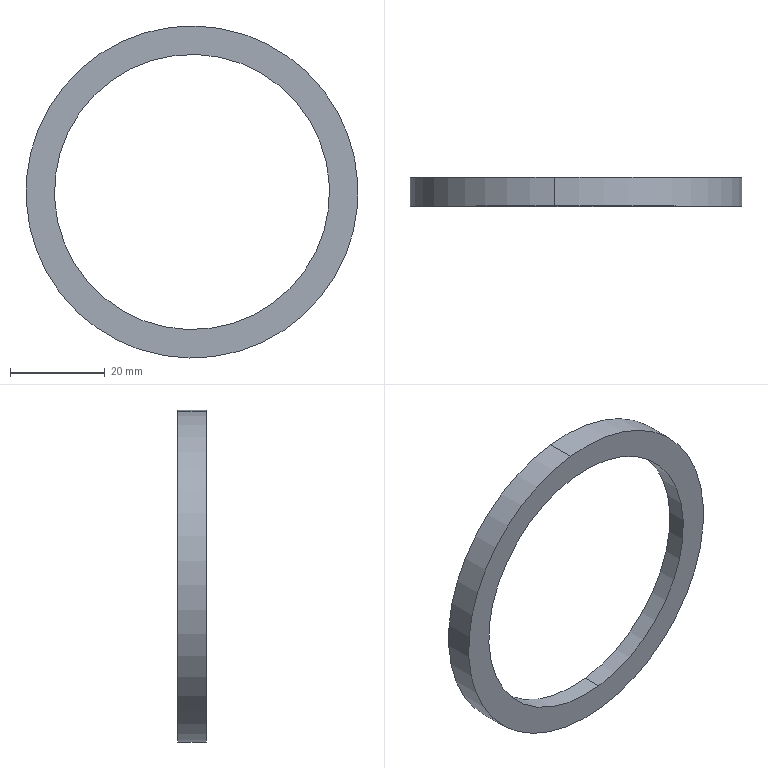Component | SolidWorks | Assembly4.1-1_118.1-1 | 1 solid | 9 faces | box 70 x 6 x 70 mm | volume 6088 mm3 | cylinder 6 | plane 3 | commonest cylinder face diameters 64 x2 70 x2 58 x2
build123d program:
from build123d import *

# Parameters (mm, degrees)
SKETCH1_R           = 35
SKETCH1_R_2         = 29
BOSS_EXTRUDE1_DEPTH = 6
SKETCH2_R           = 32
CUT_EXTRUDE1_DEPTH  = 2


with BuildPart() as part:
    # Sketch1 → Boss-Extrude1 (new body)
    with BuildSketch(Plane.XY):
        Circle(SKETCH1_R)
        Circle(SKETCH1_R_2, mode=Mode.SUBTRACT)
    extrude(amount=BOSS_EXTRUDE1_DEPTH)

    # Sketch2 → Cut-Extrude1 (cut)
    with BuildSketch(Plane.XY.offset(6)):
        Circle(SKETCH2_R)
    extrude(amount=-CUT_EXTRUDE1_DEPTH, mode=Mode.SUBTRACT)


solid = part.part

# Placed as in the assembly
solid = solid.moved(Location((0, -39.5, -0.4), (-90, 0, 0)))
STEP:
#1=COLOUR_RGB('',0.7922,0.8196,0.9333);
#2=FILL_AREA_STYLE_COLOUR('',#1);
#3=FILL_AREA_STYLE('',(#2));
#4=SURFACE_STYLE_FILL_AREA(#3);
#5=SURFACE_SIDE_STYLE('',(#4));
#6=SURFACE_STYLE_USAGE(.BOTH.,#5);
#7=PRESENTATION_STYLE_ASSIGNMENT((#6));
#8=CARTESIAN_POINT('',(-0.1653,-1.398,1.233));
#9=VERTEX_POINT('',#8);
#10=CARTESIAN_POINT('',(0.1653,-1.398,-1.265));
#11=VERTEX_POINT('',#10);
#12=CARTESIAN_POINT('',(-0.,-1.398,-0.01575));
#13=DIRECTION('',(0.,1.,-0.));
#14=DIRECTION('',(0.1312,0.,-0.9914));
#15=AXIS2_PLACEMENT_3D('',#12,#13,#14);
#16=CIRCLE('',#15,1.26);
#17=EDGE_CURVE('',#9,#11,#16,.T.);
#18=ORIENTED_EDGE('',*,*,#17,.F.);
#19=CARTESIAN_POINT('',(-0.1653,-1.319,1.233));
#20=VERTEX_POINT('',#19);
#21=CARTESIAN_POINT('',(-0.1653,-1.398,1.233));
#22=DIRECTION('',(0.,1.,-0.));
#23=VECTOR('',#22,39.37);
#24=LINE('',#21,#23);
#25=EDGE_CURVE('',#9,#20,#24,.T.);
#26=ORIENTED_EDGE('',*,*,#25,.T.);
#27=CARTESIAN_POINT('',(0.1653,-1.319,-1.265));
#28=VERTEX_POINT('',#27);
#29=CARTESIAN_POINT('',(-0.,-1.319,-0.01575));
#30=DIRECTION('',(0.,1.,-0.));
#31=DIRECTION('',(0.1312,0.,-0.9914));
#32=AXIS2_PLACEMENT_3D('',#29,#30,#31);
#33=CIRCLE('',#32,1.26);
#34=EDGE_CURVE('',#20,#28,#33,.T.);
#35=ORIENTED_EDGE('',*,*,#34,.T.);
#36=CARTESIAN_POINT('',(0.1653,-1.398,-1.265));
#37=DIRECTION('',(0.,1.,-0.));
#38=VECTOR('',#37,39.37);
#39=LINE('',#36,#38);
#40=EDGE_CURVE('',#11,#28,#39,.T.);
#41=ORIENTED_EDGE('',*,*,#40,.F.);
#42=EDGE_LOOP('',(#18,#26,#35,#41));
#43=FACE_OUTER_BOUND('',#42,.T.);
#44=CARTESIAN_POINT('',(-0.,-1.398,-0.01575));
#45=DIRECTION('',(0.,1.,-0.));
#46=DIRECTION('',(0.1312,0.,-0.9914));
#47=AXIS2_PLACEMENT_3D('',#44,#45,#46);
#48=CYLINDRICAL_SURFACE('',#47,1.26);
#49=ADVANCED_FACE('',(#43),#48,.F.);
#50=CARTESIAN_POINT('',(0.1808,-1.319,-1.382));
#51=VERTEX_POINT('',#50);
#52=CARTESIAN_POINT('',(-0.1808,-1.319,1.35));
#53=VERTEX_POINT('',#52);
#54=CARTESIAN_POINT('',(-0.,-1.319,-0.01575));
#55=DIRECTION('',(0.,1.,-0.));
#56=DIRECTION('',(0.1312,0.,-0.9914));
#57=AXIS2_PLACEMENT_3D('',#54,#55,#56);
#58=CIRCLE('',#57,1.378);
#59=EDGE_CURVE('',#51,#53,#58,.T.);
#60=ORIENTED_EDGE('',*,*,#59,.F.);
#61=CARTESIAN_POINT('',(0.1808,-1.555,-1.382));
#62=VERTEX_POINT('',#61);
#63=CARTESIAN_POINT('',(0.1808,-1.319,-1.382));
#64=DIRECTION('',(-0.,-1.,0.));
#65=VECTOR('',#64,39.37);
#66=LINE('',#63,#65);
#67=EDGE_CURVE('',#51,#62,#66,.T.);
#68=ORIENTED_EDGE('',*,*,#67,.T.);
#69=CARTESIAN_POINT('',(-0.1808,-1.555,1.35));
#70=VERTEX_POINT('',#69);
#71=CARTESIAN_POINT('',(-0.,-1.555,-0.01575));
#72=DIRECTION('',(0.,1.,-0.));
#73=DIRECTION('',(0.1312,0.,-0.9914));
#74=AXIS2_PLACEMENT_3D('',#71,#72,#73);
#75=CIRCLE('',#74,1.378);
#76=EDGE_CURVE('',#62,#70,#75,.T.);
#77=ORIENTED_EDGE('',*,*,#76,.T.);
#78=CARTESIAN_POINT('',(-0.1808,-1.319,1.35));
#79=DIRECTION('',(-0.,-1.,0.));
#80=VECTOR('',#79,39.37);
#81=LINE('',#78,#80);
#82=EDGE_CURVE('',#53,#70,#81,.T.);
#83=ORIENTED_EDGE('',*,*,#82,.F.);
#84=EDGE_LOOP('',(#60,#68,#77,#83));
#85=FACE_OUTER_BOUND('',#84,.T.);
#86=CARTESIAN_POINT('',(-0.,-1.319,-0.01575));
#87=DIRECTION('',(-0.,-1.,0.));
#88=DIRECTION('',(-0.1312,0.,0.9914));
#89=AXIS2_PLACEMENT_3D('',#86,#87,#88);
#90=CYLINDRICAL_SURFACE('',#89,1.378);
#91=ADVANCED_FACE('',(#85),#90,.T.);
#92=CARTESIAN_POINT('',(-0.1498,-1.398,1.116));
#93=VERTEX_POINT('',#92);
#94=CARTESIAN_POINT('',(0.1498,-1.398,-1.148));
#95=VERTEX_POINT('',#94);
#96=CARTESIAN_POINT('',(-0.,-1.398,-0.01575));
#97=DIRECTION('',(0.,1.,-0.));
#98=DIRECTION('',(0.1312,0.,-0.9914));
#99=AXIS2_PLACEMENT_3D('',#96,#97,#98);
#100=CIRCLE('',#99,1.142);
#101=EDGE_CURVE('',#93,#95,#100,.T.);
#102=ORIENTED_EDGE('',*,*,#101,.T.);
#103=CARTESIAN_POINT('',(0.1498,-1.555,-1.148));
#104=VERTEX_POINT('',#103);
#105=CARTESIAN_POINT('',(0.1498,-1.319,-1.148));
#106=DIRECTION('',(-0.,-1.,0.));
#107=VECTOR('',#106,39.37);
#108=LINE('',#105,#107);
#109=EDGE_CURVE('',#95,#104,#108,.T.);
#110=ORIENTED_EDGE('',*,*,#109,.T.);
#111=CARTESIAN_POINT('',(-0.1498,-1.555,1.116));
#112=VERTEX_POINT('',#111);
#113=CARTESIAN_POINT('',(-0.,-1.555,-0.01575));
#114=DIRECTION('',(0.,1.,-0.));
#115=DIRECTION('',(0.1312,0.,-0.9914));
#116=AXIS2_PLACEMENT_3D('',#113,#114,#115);
#117=CIRCLE('',#116,1.142);
#118=EDGE_CURVE('',#112,#104,#117,.T.);
#119=ORIENTED_EDGE('',*,*,#118,.F.);
#120=CARTESIAN_POINT('',(-0.1498,-1.319,1.116));
#121=DIRECTION('',(-0.,-1.,0.));
#122=VECTOR('',#121,39.37);
#123=LINE('',#120,#122);
#124=EDGE_CURVE('',#93,#112,#123,.T.);
#125=ORIENTED_EDGE('',*,*,#124,.F.);
#126=EDGE_LOOP('',(#102,#110,#119,#125));
#127=FACE_OUTER_BOUND('',#126,.T.);
#128=CARTESIAN_POINT('',(-0.,-1.319,-0.01575));
#129=DIRECTION('',(-0.,-1.,0.));
#130=DIRECTION('',(-0.1312,0.,0.9914));
#131=AXIS2_PLACEMENT_3D('',#128,#129,#130);
#132=CYLINDRICAL_SURFACE('',#131,1.142);
#133=ADVANCED_FACE('',(#127),#132,.F.);
#134=ORIENTED_EDGE('',*,*,#109,.F.);
#135=CARTESIAN_POINT('',(-0.,-1.398,-0.01575));
#136=DIRECTION('',(0.,1.,-0.));
#137=DIRECTION('',(0.1312,0.,-0.9914));
#138=AXIS2_PLACEMENT_3D('',#135,#136,#137);
#139=CIRCLE('',#138,1.142);
#140=EDGE_CURVE('',#95,#93,#139,.T.);
#141=ORIENTED_EDGE('',*,*,#140,.T.);
#142=ORIENTED_EDGE('',*,*,#124,.T.);
#143=CARTESIAN_POINT('',(-0.,-1.555,-0.01575));
#144=DIRECTION('',(0.,1.,-0.));
#145=DIRECTION('',(0.1312,0.,-0.9914));
#146=AXIS2_PLACEMENT_3D('',#143,#144,#145);
#147=CIRCLE('',#146,1.142);
#148=EDGE_CURVE('',#104,#112,#147,.T.);
#149=ORIENTED_EDGE('',*,*,#148,.F.);
#150=EDGE_LOOP('',(#134,#141,#142,#149));
#151=FACE_OUTER_BOUND('',#150,.T.);
#152=CARTESIAN_POINT('',(-0.,-1.319,-0.01575));
#153=DIRECTION('',(-0.,-1.,0.));
#154=DIRECTION('',(-0.1312,0.,0.9914));
#155=AXIS2_PLACEMENT_3D('',#152,#153,#154);
#156=CYLINDRICAL_SURFACE('',#155,1.142);
#157=ADVANCED_FACE('',(#151),#156,.F.);
#158=CARTESIAN_POINT('',(-0.,-1.319,-0.01575));
#159=DIRECTION('',(0.,1.,-0.));
#160=DIRECTION('',(0.1312,0.,-0.9914));
#161=AXIS2_PLACEMENT_3D('',#158,#159,#160);
#162=CIRCLE('',#161,1.26);
#163=EDGE_CURVE('',#28,#20,#162,.T.);
#164=ORIENTED_EDGE('',*,*,#163,.F.);
#165=ORIENTED_EDGE('',*,*,#34,.F.);
#166=EDGE_LOOP('',(#164,#165));
#167=FACE_BOUND('',#166,.T.);
#168=CARTESIAN_POINT('',(-0.,-1.319,-0.01575));
#169=DIRECTION('',(0.,1.,-0.));
#170=DIRECTION('',(0.1312,0.,-0.9914));
#171=AXIS2_PLACEMENT_3D('',#168,#169,#170);
#172=CIRCLE('',#171,1.378);
#173=EDGE_CURVE('',#53,#51,#172,.T.);
#174=ORIENTED_EDGE('',*,*,#173,.T.);
#175=ORIENTED_EDGE('',*,*,#59,.T.);
#176=EDGE_LOOP('',(#174,#175));
#177=FACE_OUTER_BOUND('',#176,.T.);
#178=CARTESIAN_POINT('',(-0.,-1.319,-0.01575));
#179=DIRECTION('',(0.,1.,-0.));
#180=DIRECTION('',(0.1312,-0.,-0.9914));
#181=AXIS2_PLACEMENT_3D('',#178,#179,#180);
#182=PLANE('',#181);
#183=ADVANCED_FACE('',(#167,#177),#182,.T.);
#184=CARTESIAN_POINT('',(-0.,-1.555,-0.01575));
#185=DIRECTION('',(0.,1.,-0.));
#186=DIRECTION('',(0.1312,0.,-0.9914));
#187=AXIS2_PLACEMENT_3D('',#184,#185,#186);
#188=CIRCLE('',#187,1.378);
#189=EDGE_CURVE('',#70,#62,#188,.T.);
#190=ORIENTED_EDGE('',*,*,#189,.F.);
#191=ORIENTED_EDGE('',*,*,#76,.F.);
#192=EDGE_LOOP('',(#190,#191));
#193=FACE_OUTER_BOUND('',#192,.T.);
#194=ORIENTED_EDGE('',*,*,#118,.T.);
#195=ORIENTED_EDGE('',*,*,#148,.T.);
#196=EDGE_LOOP('',(#194,#195));
#197=FACE_BOUND('',#196,.T.);
#198=CARTESIAN_POINT('',(-0.,-1.555,-0.01575));
#199=DIRECTION('',(0.,1.,-0.));
#200=DIRECTION('',(0.1312,-0.,-0.9914));
#201=AXIS2_PLACEMENT_3D('',#198,#199,#200);
#202=PLANE('',#201);
#203=ADVANCED_FACE('',(#193,#197),#202,.F.);
#204=ORIENTED_EDGE('',*,*,#67,.F.);
#205=ORIENTED_EDGE('',*,*,#173,.F.);
#206=ORIENTED_EDGE('',*,*,#82,.T.);
#207=ORIENTED_EDGE('',*,*,#189,.T.);
#208=EDGE_LOOP('',(#204,#205,#206,#207));
#209=FACE_OUTER_BOUND('',#208,.T.);
#210=CARTESIAN_POINT('',(-0.,-1.319,-0.01575));
#211=DIRECTION('',(-0.,-1.,0.));
#212=DIRECTION('',(-0.1312,0.,0.9914));
#213=AXIS2_PLACEMENT_3D('',#210,#211,#212);
#214=CYLINDRICAL_SURFACE('',#213,1.378);
#215=ADVANCED_FACE('',(#209),#214,.T.);
#216=ORIENTED_EDGE('',*,*,#25,.F.);
#217=CARTESIAN_POINT('',(-0.,-1.398,-0.01575));
#218=DIRECTION('',(0.,1.,-0.));
#219=DIRECTION('',(0.1312,0.,-0.9914));
#220=AXIS2_PLACEMENT_3D('',#217,#218,#219);
#221=CIRCLE('',#220,1.26);
#222=EDGE_CURVE('',#11,#9,#221,.T.);
#223=ORIENTED_EDGE('',*,*,#222,.F.);
#224=ORIENTED_EDGE('',*,*,#40,.T.);
#225=ORIENTED_EDGE('',*,*,#163,.T.);
#226=EDGE_LOOP('',(#216,#223,#224,#225));
#227=FACE_OUTER_BOUND('',#226,.T.);
#228=CARTESIAN_POINT('',(-0.,-1.398,-0.01575));
#229=DIRECTION('',(0.,1.,-0.));
#230=DIRECTION('',(0.1312,0.,-0.9914));
#231=AXIS2_PLACEMENT_3D('',#228,#229,#230);
#232=CYLINDRICAL_SURFACE('',#231,1.26);
#233=ADVANCED_FACE('',(#227),#232,.F.);
#234=ORIENTED_EDGE('',*,*,#101,.F.);
#235=ORIENTED_EDGE('',*,*,#140,.F.);
#236=EDGE_LOOP('',(#234,#235));
#237=FACE_BOUND('',#236,.T.);
#238=ORIENTED_EDGE('',*,*,#222,.T.);
#239=ORIENTED_EDGE('',*,*,#17,.T.);
#240=EDGE_LOOP('',(#238,#239));
#241=FACE_OUTER_BOUND('',#240,.T.);
#242=CARTESIAN_POINT('',(-0.,-1.398,-0.01575));
#243=DIRECTION('',(0.,1.,-0.));
#244=DIRECTION('',(0.1312,-0.,-0.9914));
#245=AXIS2_PLACEMENT_3D('',#242,#243,#244);
#246=PLANE('',#245);
#247=ADVANCED_FACE('',(#237,#241),#246,.T.);
#248=CLOSED_SHELL('',(#49,#91,#133,#157,#183,#203,#215,#233,#247));
#249=MANIFOLD_SOLID_BREP('',#248);
#250=STYLED_ITEM('',(#7),#249);
#251=PRESENTATION_LAYER_ASSIGNMENT('','',(#250));
#252=(LENGTH_UNIT()NAMED_UNIT(*)SI_UNIT($,.METRE.));
#253=LENGTH_MEASURE_WITH_UNIT(LENGTH_MEASURE(0.0254),#252);
#254=DIMENSIONAL_EXPONENTS(1.,0.,0.,0.,0.,0.,0.);
#255=(CONVERSION_BASED_UNIT('',#253)LENGTH_UNIT()NAMED_UNIT(#254));
#256=UNCERTAINTY_MEASURE_WITH_UNIT(LENGTH_MEASURE(0.00001),#255,'','');
#257=(NAMED_UNIT(*)PLANE_ANGLE_UNIT()SI_UNIT($,.RADIAN.));
#258=(NAMED_UNIT(*)SI_UNIT($,.STERADIAN.)SOLID_ANGLE_UNIT());
#259=(GEOMETRIC_REPRESENTATION_CONTEXT(3)GLOBAL_UNCERTAINTY_ASSIGNED_CONTEXT((#256))GLOBAL_UNIT_ASSIGNED_CONTEXT((#255,#257,#258))REPRESENTATION_CONTEXT('',''));
#260=MECHANICAL_DESIGN_GEOMETRIC_PRESENTATION_REPRESENTATION('',(#250),#259);
#261=CARTESIAN_POINT('',(0.,0.,0.));
#262=DIRECTION('',(0.,0.,1.));
#263=DIRECTION('',(1.,0.,0.));
#264=AXIS2_PLACEMENT_3D('',#261,#262,#263);
#265=(LENGTH_UNIT()NAMED_UNIT(*)SI_UNIT($,.METRE.));
#266=LENGTH_MEASURE_WITH_UNIT(LENGTH_MEASURE(0.0254),#265);
#267=DIMENSIONAL_EXPONENTS(1.,0.,0.,0.,0.,0.,0.);
#268=(CONVERSION_BASED_UNIT('',#266)LENGTH_UNIT()NAMED_UNIT(#267));
#269=UNCERTAINTY_MEASURE_WITH_UNIT(LENGTH_MEASURE(0.00001),#268,'','');
#270=(NAMED_UNIT(*)PLANE_ANGLE_UNIT()SI_UNIT($,.RADIAN.));
#271=(NAMED_UNIT(*)SI_UNIT($,.STERADIAN.)SOLID_ANGLE_UNIT());
#272=(GEOMETRIC_REPRESENTATION_CONTEXT(3)GLOBAL_UNCERTAINTY_ASSIGNED_CONTEXT((#269))GLOBAL_UNIT_ASSIGNED_CONTEXT((#268,#270,#271))REPRESENTATION_CONTEXT('',''));
#273=ADVANCED_BREP_SHAPE_REPRESENTATION('',(#249,#264),#272);